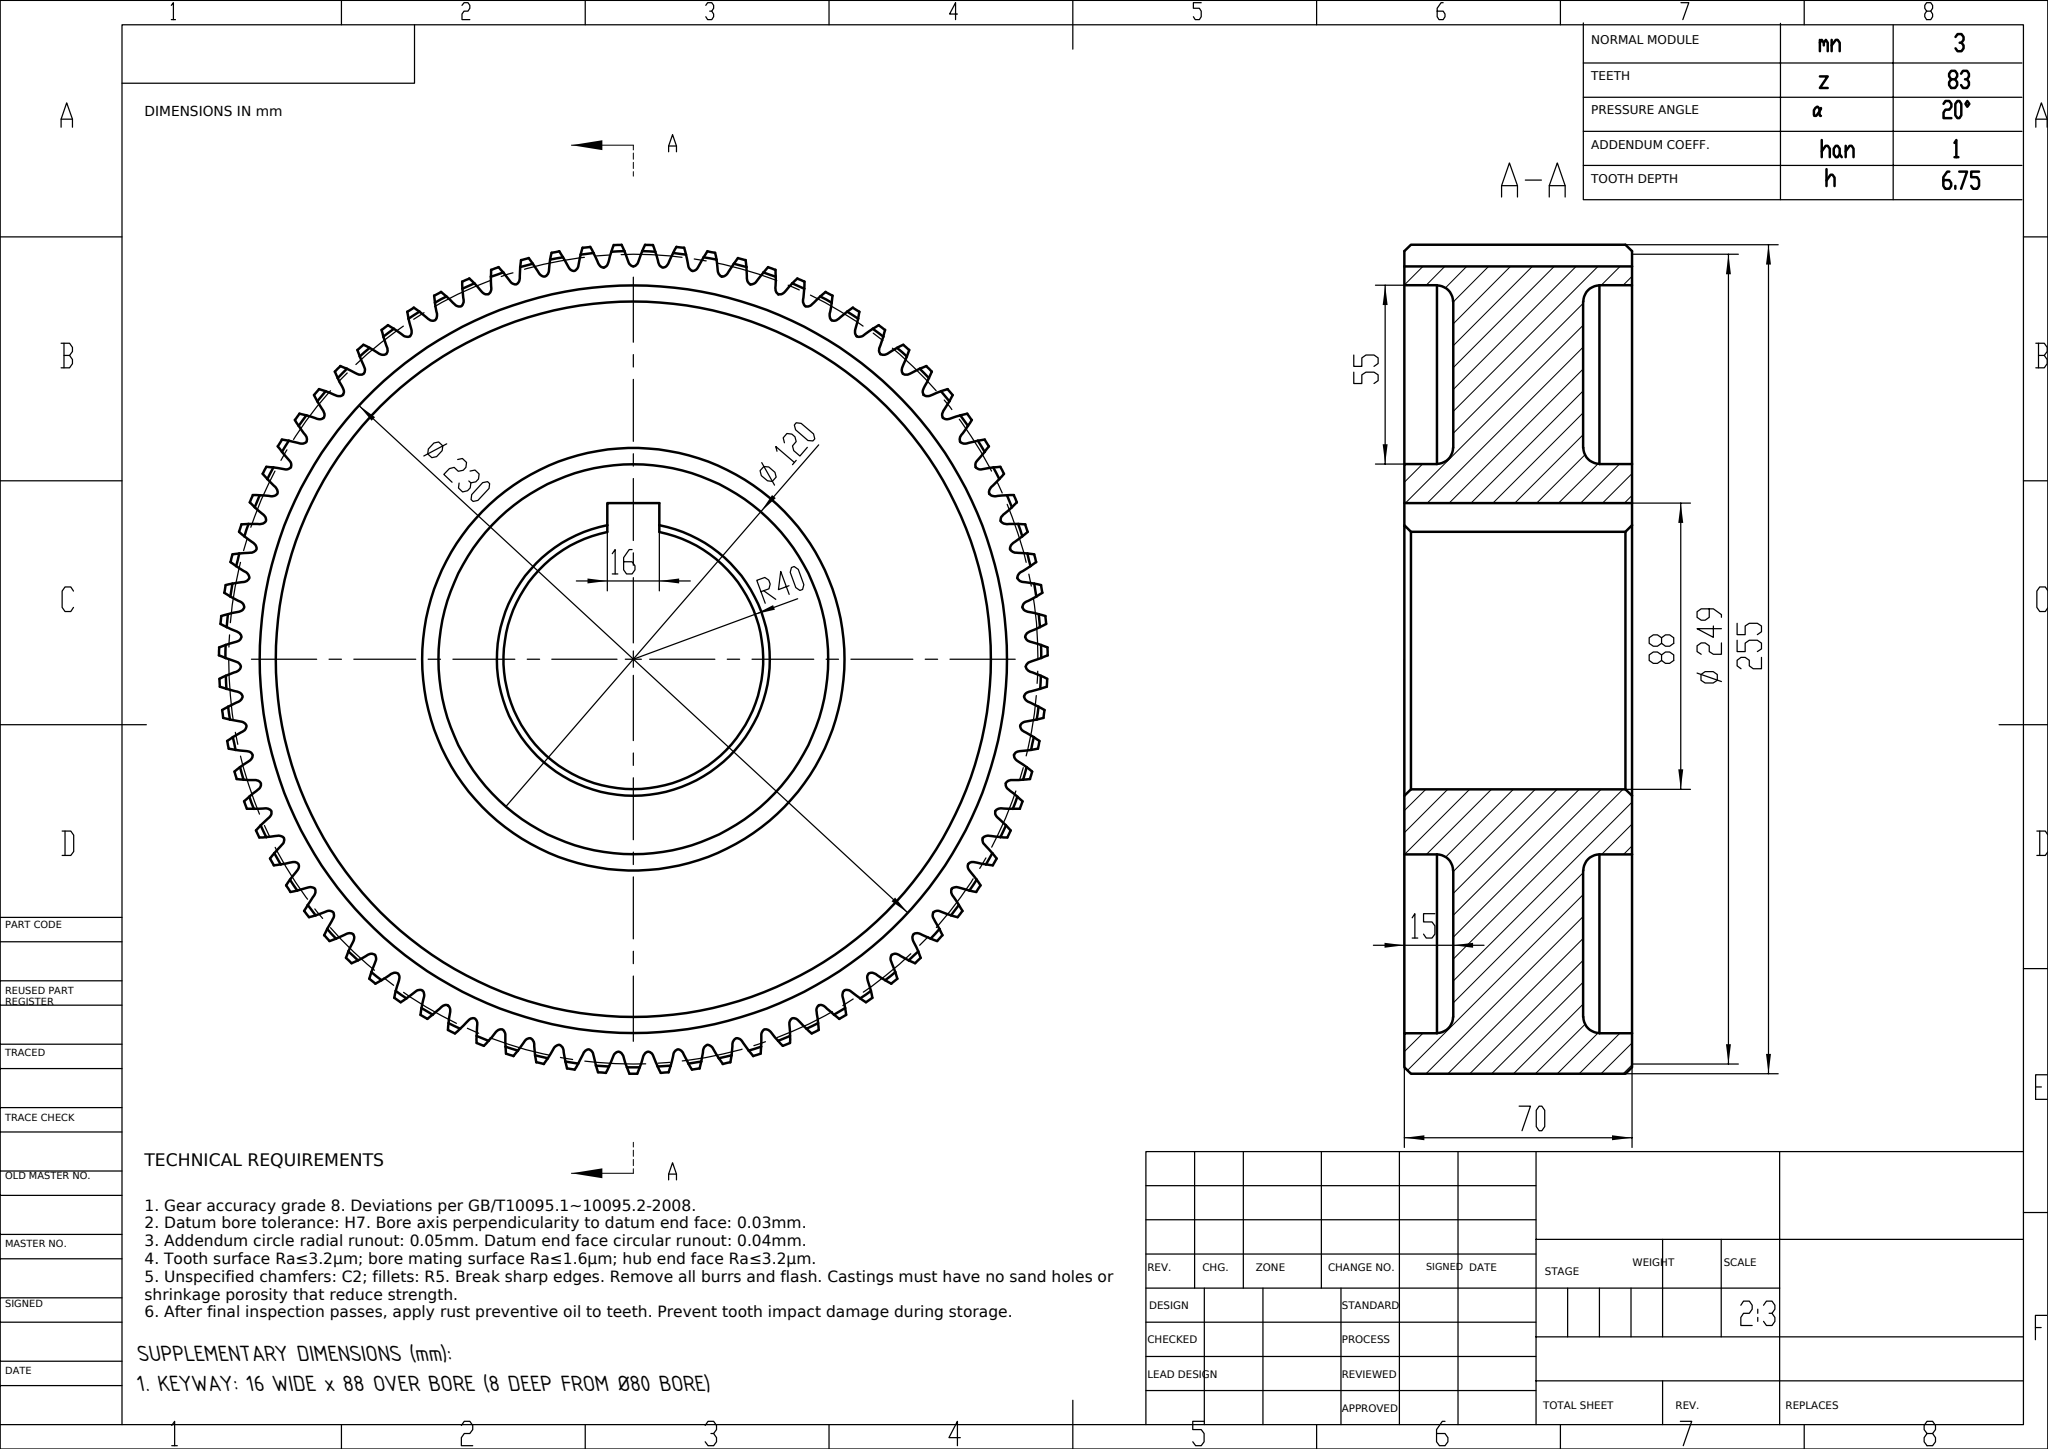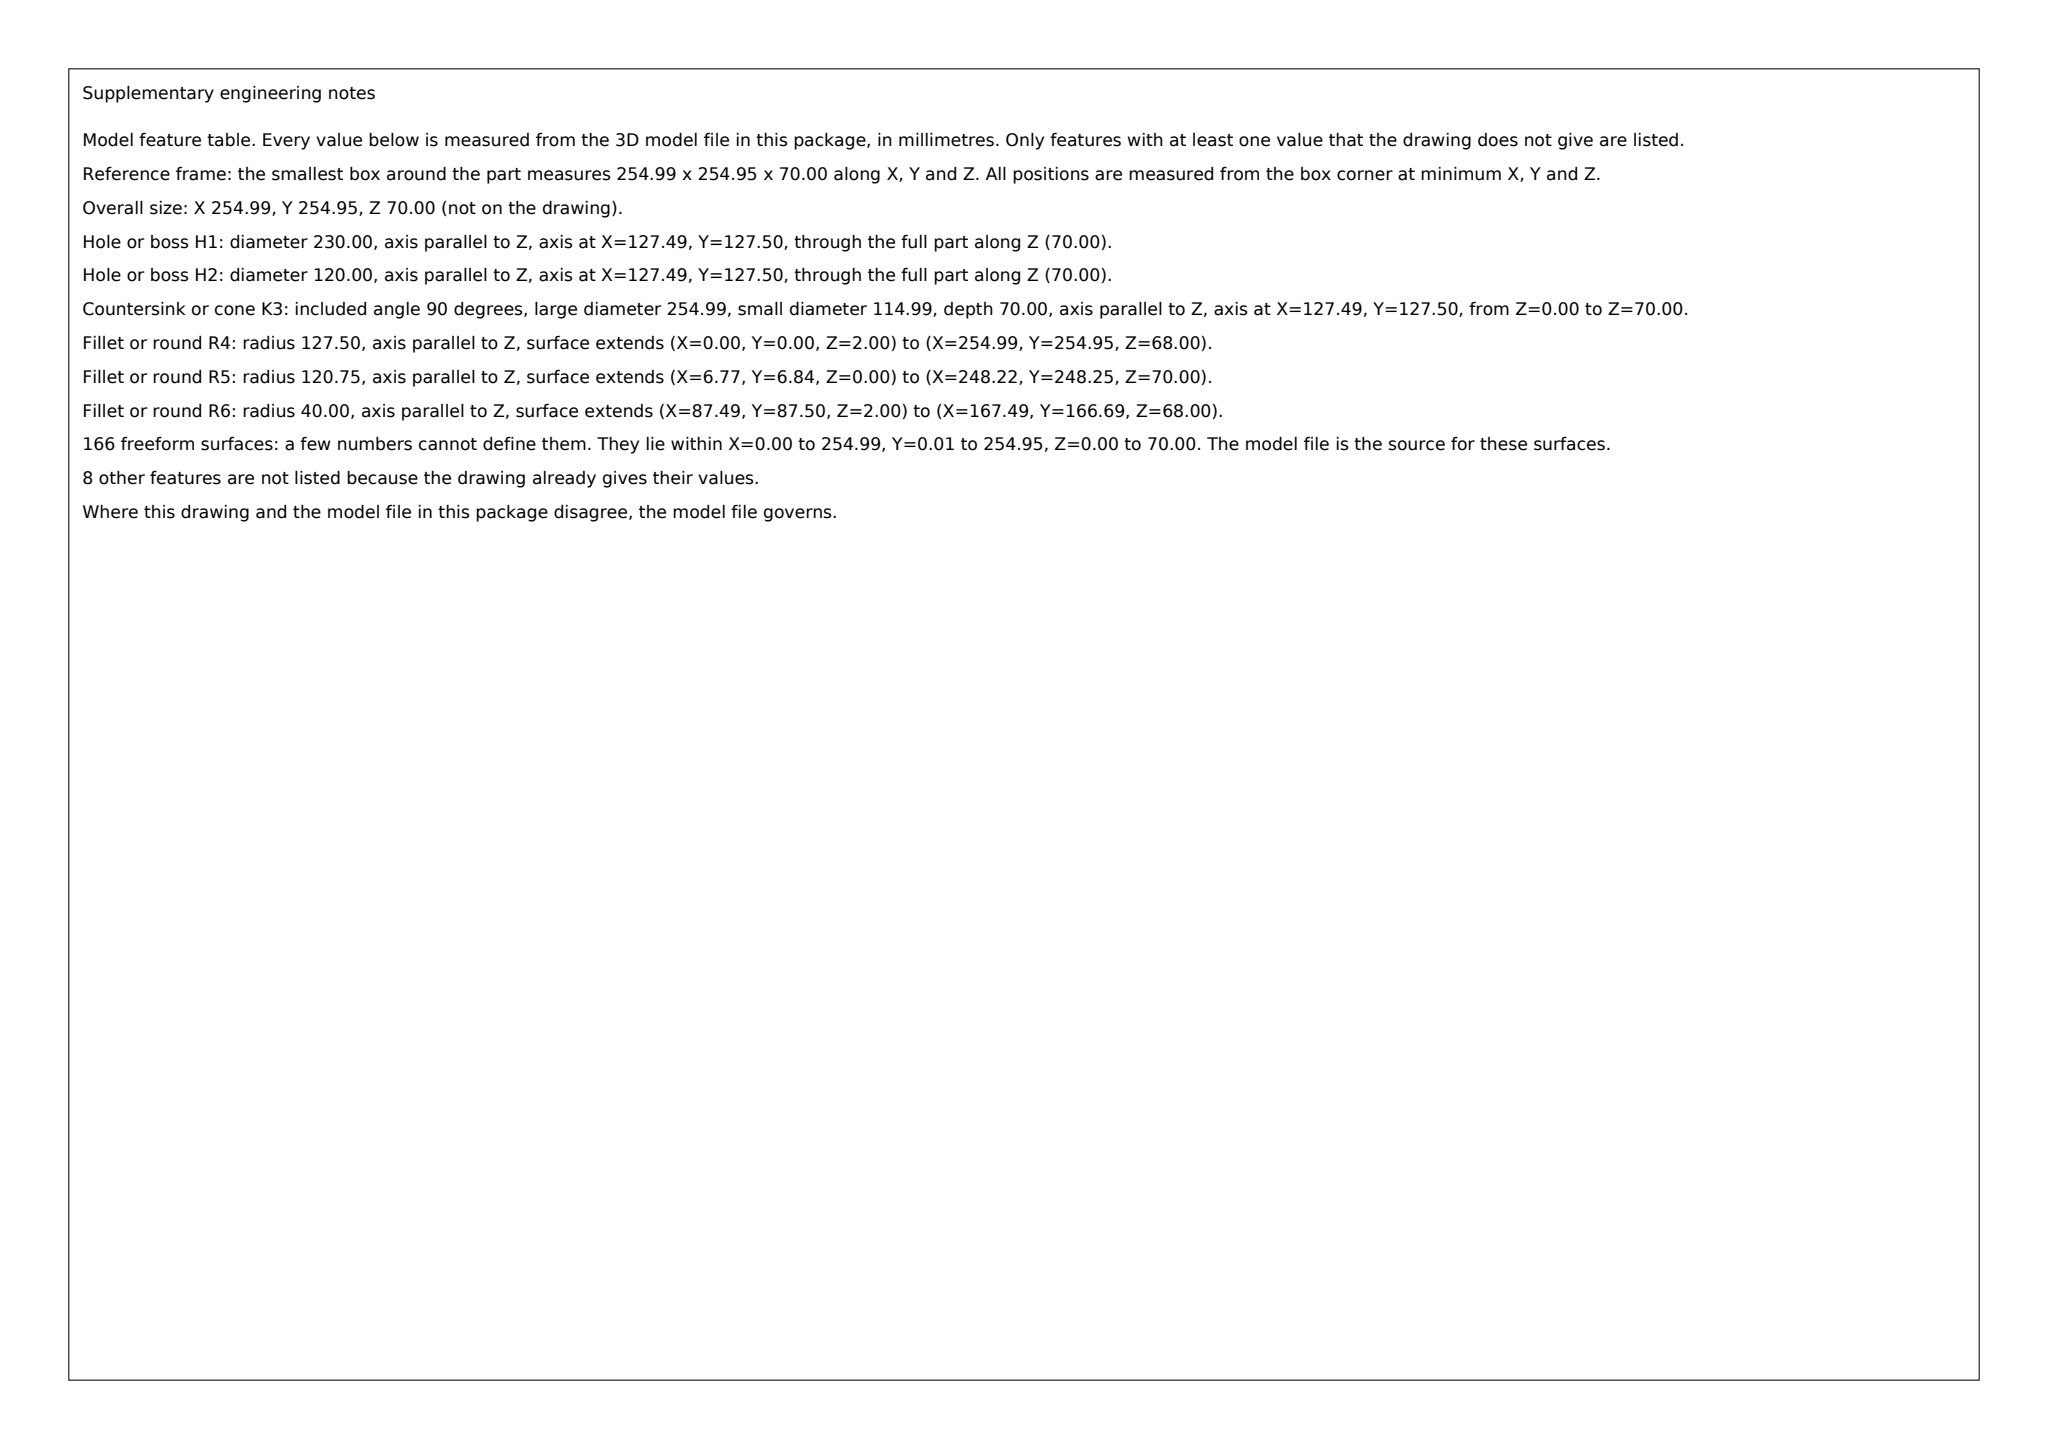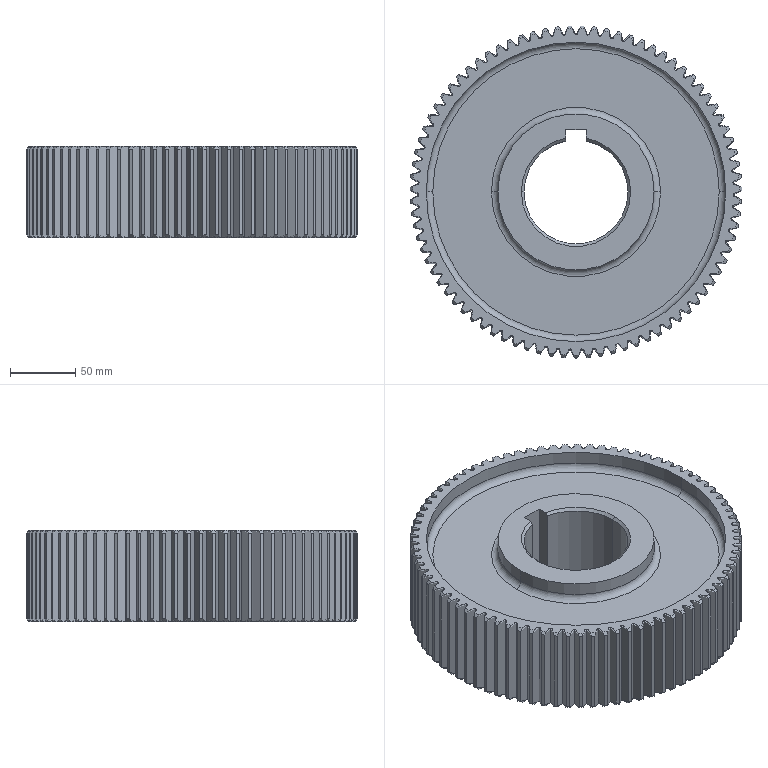Part | SolidWorks | mm | 1 solid | 532 faces | box 254.99 x 254.95 x 70 mm | volume 2147136 mm3 | cylinder 177 | cone 172 | spline 166 | plane 9 | torus 8 | commonest cylinder face diameters 255 x83 241.497 x83 120 x4 230 x4 80 x3